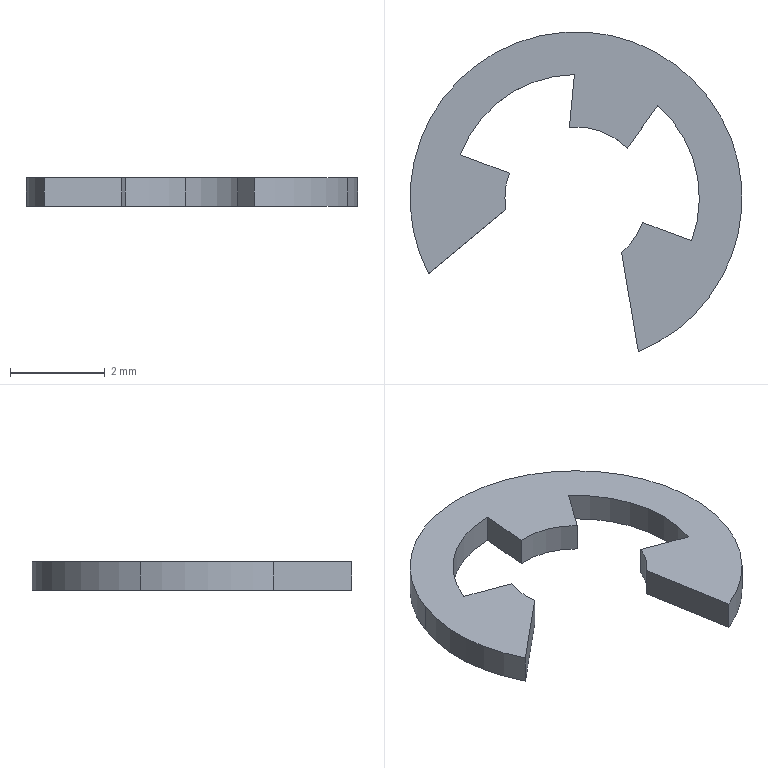Component | SolidWorks | 4ExternalCaliper-3 | 1 solid | 16 faces | volume 11 mm3 | cylinder 8 | plane 8 | commonest cylinder face diameters 7 x3 3 x3 5.2 x2